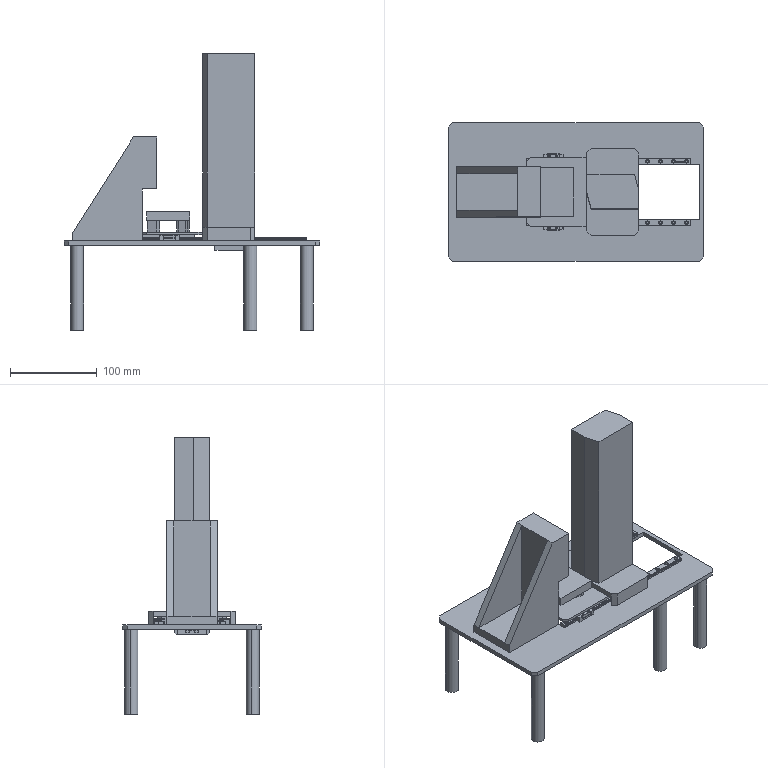Assembly | SolidWorks | mm | 21 component files | 21 solids | 1533 faces | box 295 x 160 x 319 mm | volume 1129561 mm3 | plane 955 | cylinder 332 | spline 170 | cone 76 | commonest cylinder face diameters 4.2 x58 2.4 x52 0.6 x36 2 x36 1.6 x32 15 x24 1.4 x18 1.2 x16
Bill of materials:
2023-12-12-23 | 1 | AL6061 | Tall straight prism; its cross-section is a rectangle with two diagonally opposite corners chamfered.
2023-12-12-24 | 1 | S45C | Rectangular plate with chamfered corners and a downward leg at each short end, giving a bridge or upside-down channel shape. It has two notched, irregular through-cutouts placed diagonally across from each other.
2023-12-12-25 | 1 | S45C | Thin flat plate with small chamfered corners and a large rectangular window. The window is off-center toward one end and leaves only a very thin strip at that edge.
2023-12-12-27 | 1 | S45C | Thin rectangular plate with chamfered corners and two notched, irregular through-cutouts. A rectangular block with chamfered lower corners hangs down from the underside near one end.
2023-12-12-28 | 1 |  | Thin L-shaped plate with chamfered outer corners. A perpendicular flange runs along one end edge and sticks out both above and below the plate, giving a T-shaped side profile.
2023-12-12-29 | 1 | AL6061 | Solid block with a stepped wedge profile: one long sloped face, a flat top, and a rectangular step notch on the side opposite the slope.
2023-12-12-30 | 1 | S45C | Thick square plate with two rectangular legs or posts underneath. One leg has an angled or chamfered lower section.
2023-12-12-31 | 6 |  | Plain solid cylinder, several times longer than its diameter, with flat ends.
LinearGuideMGN7(HIWIN) | 2 | Chrome Stainless Steel | Long straight rail with a single row of evenly spaced counterbored through-holes along its top. Its cross-section has chamfered top corners, round grooves on both sides and a small notch in the base.
SliderMGN7C(HIWIN) | 4 | Gray Cast Iron | Rectangular block with a channel in the underside sized to straddle a rail. It has four holes in the top in a rectangular pattern, separate end sections with seam lines, and a small hole in the end face.
TCM-10x15-0_15fp | 1 |  | Rectangular bar with three parallel cylindrical rods sticking out perpendicular to one face. The middle rod ends in a wider cylindrical section. Two small through-holes in the bar are partly cut, giving them a D shape.
TC-M-10x1515_b | 1 |  | Rectangular block with a lengthwise groove on top, two vertical through-holes, and a shallow recess with chamfered edges across the top. Each end face has four chamfered or counterbored holes, two small holes, and two keyhole-shaped slots open to the bottom edge.
Mates:
1. coincident | 2023-12-12-23-1 face at (1.222, -2.867, 100) dir (0, 0, -1) | 2023-12-12-24-1 face at (1.222, -2.867, 100) dir (0, 0, 1)
2. distance | 2023-12-12-25-1 face at (131.222, 77.133, 84) dir (0, 0, 1) | 2023-12-12-24-1 face at (1.222, -2.867, 94) dir (0, 0, -1)
3. distance | GuideRail-1/LinearGuideMGN7(HIWIN)-1 face at (-98.778, 29.333, 83) dir (0, 0, -1) | 2023-12-12-25-1 face at (131.222, 77.133, 84) dir (0, 0, 1)
4. distance | GuideRail-2/LinearGuideMGN7(HIWIN)-1 face at (91.222, -35.067, 83) dir (0, 0, -1) | 2023-12-12-25-1 face at (131.222, 77.133, 84) dir (0, 0, 1)
5. coincident | GuideRail-1/SliderMGN7C(HIWIN)-2 face at (-56.278, 24.133, 91) dir (0, 0, 1) | 2023-12-12-27-1 face at (31.222, 37.133, 91) dir (0, 0, -1)
6. distance | 2023-12-12-27-1 face at (-98.778, -42.867, 194) dir (-1, 0, 0) | GuideRail-1/SliderMGN7C(HIWIN)-2 face at (-78.778, 41.133, 87.2) dir (-1, 0, 0)
7. width | 2023-12-12-27-1 face at (31.222, 17.133, 84) dir (0, 1, 0) | 2023-12-12-27-1 face at (31.222, -22.867, 84) dir (0, -1, 0) | 2023-12-12-25-1 face at (101.222, 29.133, 84) dir (0, -1, 0) | 2023-12-12-25-1 face at (101.222, -34.867, 84) dir (0, 1, 0)
8. coincident | GuideRail-1/SliderMGN7C(HIWIN)-2 face at (-78.778, 41.133, 87.2) dir (-1, 0, 0) | GuideRail-2/SliderMGN7C(HIWIN)-1 face at (-78.778, -46.867, 87.2) dir (-1, 0, 0)
9. distance | 2023-12-12-27-1 face at (-98.778, -42.867, 194) dir (-1, 0, 0) | 2023-12-12-24-1 face at (-28.778, 47.133, 216.619) dir (-1, 0, 0)
10. coincident | GuideRail-1/LinearGuideMGN7(HIWIN)-1 face at (-98.778, 29.133, 85.6) dir (0, -1, 0) | 2023-12-12-25-1 face at (101.222, 29.133, 84) dir (0, -1, 0)
11. coincident | 2023-12-12-25-1 face at (101.222, -34.867, 84) dir (0, 1, 0) | GuideRail-2/LinearGuideMGN7(HIWIN)-1 face at (91.222, -34.867, 85.6) dir (0, 1, 0)
12. width | 2023-12-12-24-1 face at (31.222, 47.133, 216.619) dir (0, 1, 0) | 2023-12-12-24-1 face at (31.222, -52.867, 216.619) dir (0, -1, 0) | 2023-12-12-25-1 face at (131.222, -82.867, 84) dir (0, -1, 0) | 2023-12-12-25-1 face at (131.222, 77.133, 84) dir (0, 1, 0)
13. coincident | 2023-12-12-27-1 face at (31.222, 37.133, 91) dir (0, 0, -1) | TCM10x15S_0-2/TC-M-10x1515_b-1 face at (26.222, -9.367, 91) dir (0, 0, 1)
14. coincident | 2023-12-12-27-1 face at (26.222, 17.133, 91) dir (-1, 0, 0) | TCM10x15S_0-2/TC-M-10x1515_b-1 face at (26.222, -7.967, 76.3) dir (1, 0, 0)
15. distance | TCM10x15S_0-2/TC-M-10x1515_b-1 face at (26.222, -19.867, 91) dir (0, -1, 0) | 2023-12-12-27-1 face at (31.222, -22.867, 84) dir (0, -1, 0)
16. coincident | 2023-12-12-28-1 face at (-20.778, -21.367, 88.5) dir (1, 0, 0) | TCM10x15S_0-2/TCM-10x15-0_15fp-1 face at (-20.778, -2.867, 83.5) dir (-1, 0, 0)
17. distance | 2023-12-12-28-1 face at (-20.778, -21.367, 88.5) dir (0, -1, 0) | TCM10x15S_0-2/TCM-10x15-0_15fp-1 face at (-15.778, -19.367, 88.5) dir (0, -1, 0)
18. coincident | 2023-12-12-28-1 face at (-20.778, -21.367, 78.5) dir (0, 0, -1) | TCM10x15S_0-2/TCM-10x15-0_15fp-1 face at (-15.778, -19.367, 78.5) dir (0, 0, -1)
19. coincident | GuideRail-1/LinearGuideMGN7(HIWIN)-1 face at (-98.778, 36.133, 86.3) dir (-1, 0, 0) | 2023-12-12-25-1 face at (-98.778, -34.867, 84) dir (1, 0, 0)
20. coincident | GuideRail-1/LinearGuideMGN7(HIWIN)-1 face at (-98.778, 36.133, 86.3) dir (-1, 0, 0) | GuideRail-2/LinearGuideMGN7(HIWIN)-1 face at (-98.778, -41.867, 86.3) dir (-1, 0, 0)
21. distance | 2023-12-12-25-1 face at (-98.778, -34.867, 84) dir (1, 0, 0) | 2023-12-12-24-1 face at (-28.778, 47.133, 216.619) dir (-1, 0, 0)
22. coincident | 2023-12-12-25-1 face at (131.222, 77.133, 84) dir (0, 0, 1) | 2023-12-12-29-1 face at (-98.778, 26.133, 84) dir (0, 0, -1)
23. width | 2023-12-12-29-1 face at (-98.778, 26.133, 84) dir (0, 1, 0) | 2023-12-12-29-1 face at (-98.778, -31.867, 84) dir (0, -1, 0) | 2023-12-12-25-1 face at (131.222, -82.867, 84) dir (0, -1, 0) | 2023-12-12-25-1 face at (131.222, 77.133, 84) dir (0, 1, 0)
24. coincident | 2023-12-12-25-1 face at (-98.778, -34.867, 84) dir (1, 0, 0) | 2023-12-12-29-1 face at (-98.778, 26.133, 84) dir (1, 0, 0)
25. concentric | 2023-12-12-25-1 face at (91.222, 67.133, 81) dir (0, 0, -1) r 7.5 | 2023-12-12-31-1 face at (91.222, 67.133, 81) dir (0, 0, -1) r 7.5
26. coincident | 2023-12-12-25-1 face at (91.222, 67.133, 81) dir (0, 0, -1) | 2023-12-12-31-1 face at (91.222, 67.133, 81) dir (0, 0, 1)
27. concentric | 2023-12-12-25-1 face at (91.222, -72.867, 81) dir (0, 0, -1) r 7.5 | 2023-12-12-31-6 face at (91.222, -72.867, 81) dir (0, 0, -1) r 7.5
28. coincident | 2023-12-12-25-1 face at (91.222, -72.867, 81) dir (0, 0, -1) | 2023-12-12-31-6 face at (91.222, -72.867, 81) dir (0, 0, 1)
29. concentric | 2023-12-12-25-1 face at (26.222, -72.867, 81) dir (0, 0, -1) r 7.5 | 2023-12-12-31-5 face at (26.222, -72.867, 81) dir (0, 0, -1) r 7.5
30. concentric | 2023-12-12-25-1 face at (-173.778, -72.867, 81) dir (0, 0, -1) r 7.5 | 2023-12-12-31-4 face at (-173.778, -72.867, 81) dir (0, 0, -1) r 7.5
31. concentric | 2023-12-12-25-1 face at (-173.778, 67.133, 81) dir (0, 0, -1) r 7.5 | 2023-12-12-31-2 face at (-173.778, 67.133, 81) dir (0, 0, -1) r 7.5
32. concentric | 2023-12-12-25-1 face at (26.222, 67.133, 81) dir (0, 0, -1) r 7.5 | 2023-12-12-31-3 face at (26.222, 67.133, 81) dir (0, 0, -1) r 7.5
33. coincident | 2023-12-12-31-1 face at (91.222, 67.133, -19) dir (0, 0, -1) | 2023-12-12-31-3 edge at (26.222, 67.133, -19) dir (0, 0, 1) r 7.5
34. coincident | 2023-12-12-31-2 face at (-173.778, 67.133, -19) dir (0, 0, -1) | 2023-12-12-31-3 face at (26.222, 67.133, -19) dir (0, 0, -1)
35. coincident | 2023-12-12-31-2 face at (-173.778, 67.133, -19) dir (0, 0, -1) | 2023-12-12-31-4 face at (-173.778, -72.867, -19) dir (0, 0, -1)
36. coincident | 2023-12-12-31-4 face at (-173.778, -72.867, -19) dir (0, 0, -1) | 2023-12-12-31-5 face at (26.222, -72.867, -19) dir (0, 0, -1)
37. concentric | LinearGuideMGN7(HIWIN)-1 face at (3.232, 0.1463, -17.5) dir (0, 0, 1) r 0.7 | SliderMGN7C(HIWIN)-1 face at (3.232, 0.1463, 206.25) dir (0, 0, -1) r 0.7
38. concentric | LinearGuideMGN7(HIWIN)-1 face at (-3.768, 0.1463, -17.5) dir (0, 0, 1) r 0.7 | SliderMGN7C(HIWIN)-1 face at (-3.768, 0.1463, 206.25) dir (0, 0, -1) r 0.7
39. concentric | LinearGuideMGN7(HIWIN)-1 face at (-3.768, 0.1463, -17.5) dir (0, 0, 1) r 0.7 | SliderMGN7C(HIWIN)-2 face at (-3.768, 0.1463, 138.75) dir (0, 0, -1) r 0.7
40. concentric | LinearGuideMGN7(HIWIN)-1 face at (3.232, 0.1463, -17.5) dir (0, 0, 1) r 0.7 | SliderMGN7C(HIWIN)-2 face at (3.232, 0.1463, 138.75) dir (0, 0, -1) r 0.7
41. distance | SliderMGN7C(HIWIN)-1 face at (8.232, 1.046, 175) dir (0, 0, -1) | SliderMGN7C(HIWIN)-2 face at (8.232, 1.046, 130) dir (0, 0, 1)
42. distance | LinearGuideMGN7(HIWIN)-1 face at (3.232, 0.1463, -17.5) dir (0, 0, -1) | SliderMGN7C(HIWIN)-2 face at (8.232, 1.046, 107.5) dir (0, 0, -1)
43. distance | TCM-10x15-0_15fp-1 face at (-21, 0, 0) dir (-1, 0, 0) | TC-M-10x1515_b-1 face at (0, 5.1, 7.2) dir (-1, 0, 0)
44. concentric | TC-M-10x1515_b-1 face at (36, 0, 0) dir (-1, 0, 0) r 5.9 | TCM-10x15-0_15fp-1 face at (21, 0, 0) dir (-1, 0, 0) r 2.5
45. concentric | TC-M-10x1515_b-1 face at (41, -11.5, 0) dir (-1, 0, 0) r 3 | TCM-10x15-0_15fp-1 face at (14.5, -11.5, 0) dir (-1, 0, 0) r 3